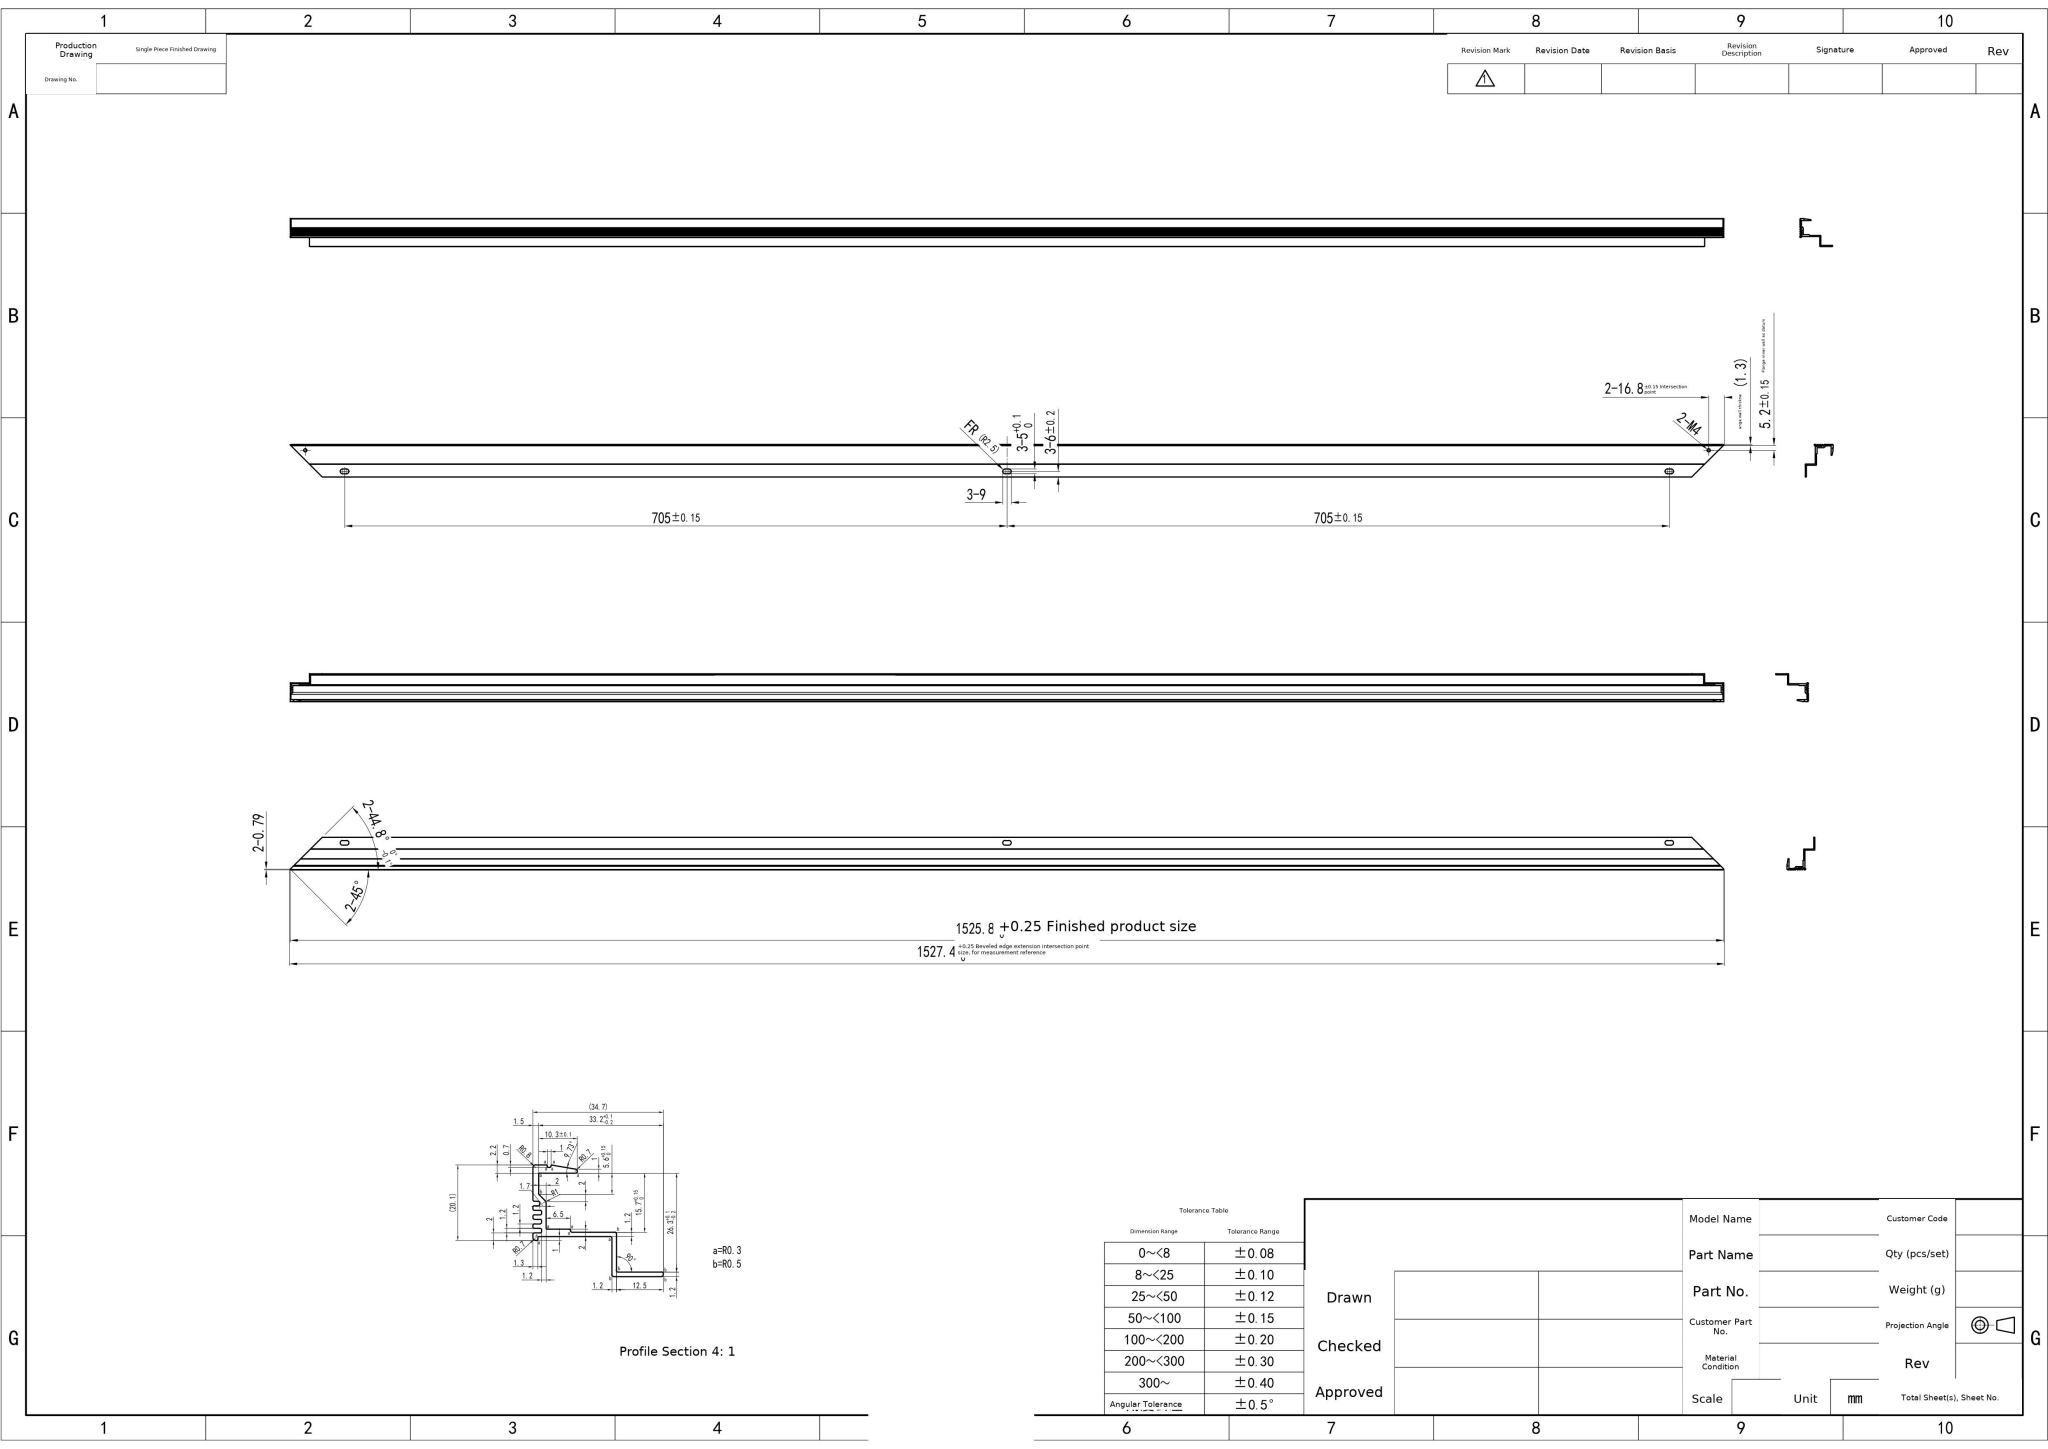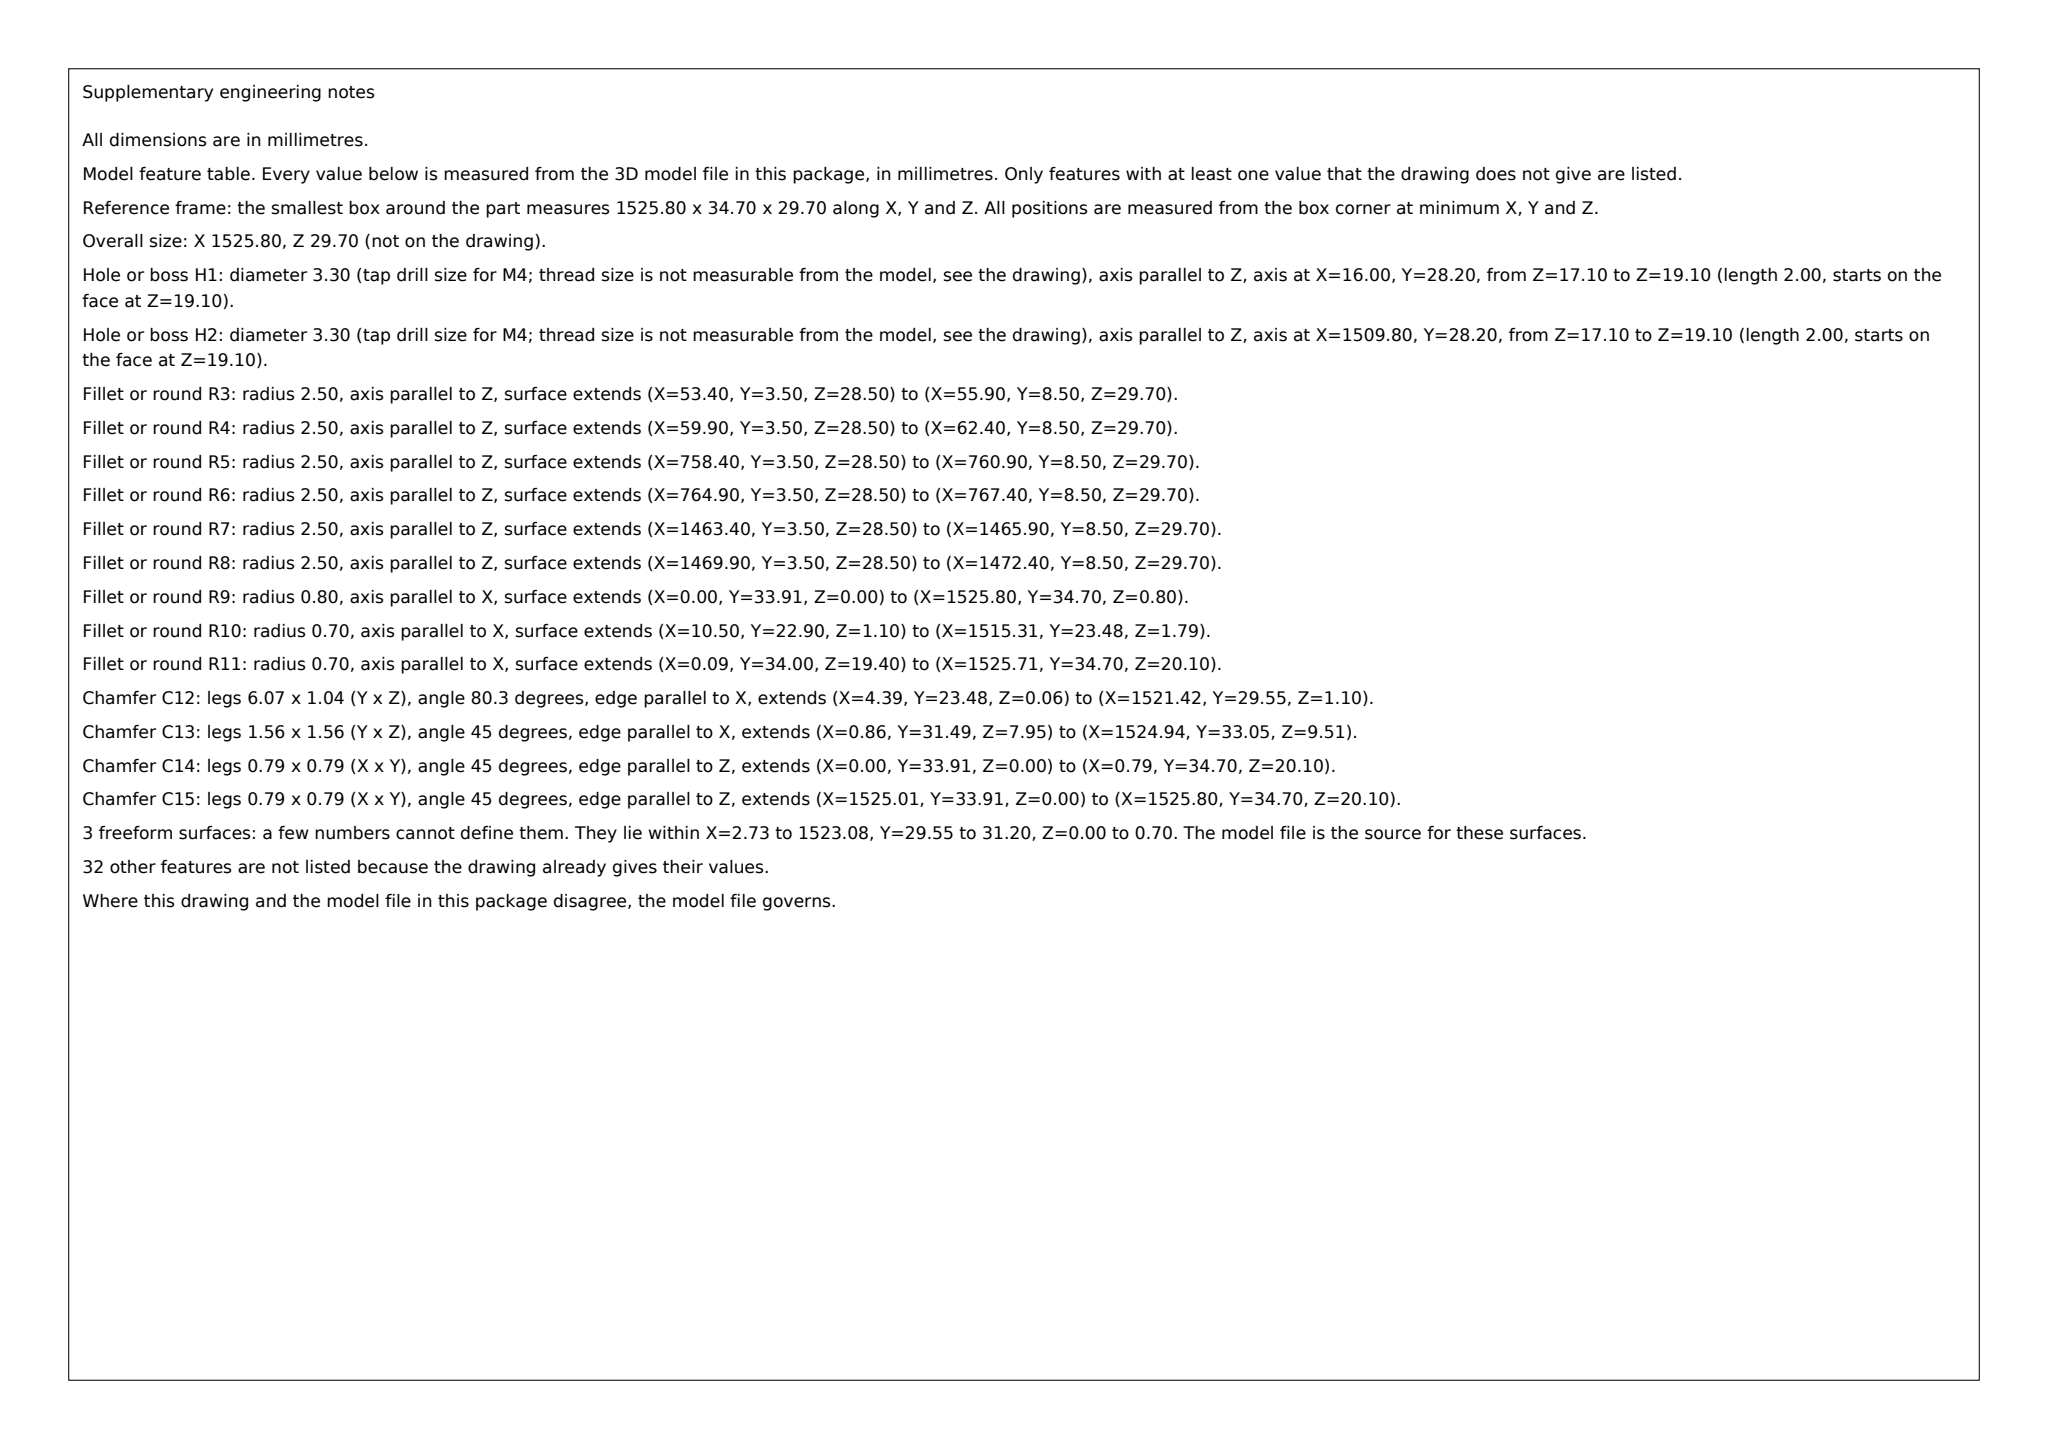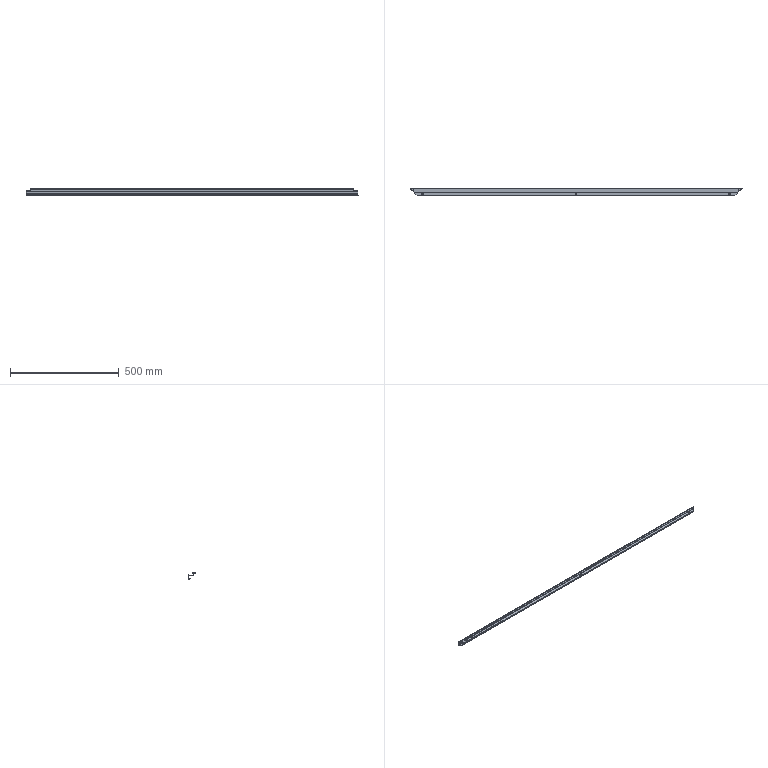Part | SolidWorks | mm | 1 solid | 106 faces | box 1525.8 x 34.7 x 29.7 mm | volume 169684 mm3 | plane 55 | cylinder 48 | spline 3 | commonest cylinder face diameters 0.8 x16 5 x9 0.6 x9 1 x6 3.3 x4 1.4 x2 1.6 x1 2 x1